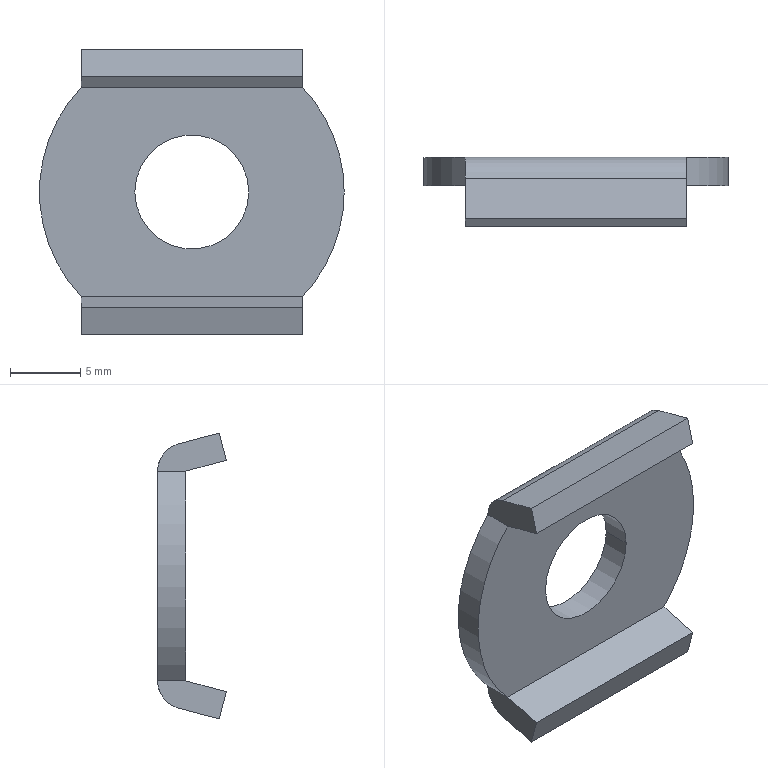Component | SolidWorks | CH-225-D-1_FW-516-1 | 1 solid | 19 faces | box 21.65 x 4.9 x 20.32 mm | volume 757 mm3 | plane 12 | cylinder 7 | commonest cylinder face diameters 21.645 x3 8.1 x2 4 x2
STEP:
#1=COLOUR_RGB('',0.7922,0.8196,0.9333);
#2=FILL_AREA_STYLE_COLOUR('',#1);
#3=FILL_AREA_STYLE('',(#2));
#4=SURFACE_STYLE_FILL_AREA(#3);
#5=SURFACE_SIDE_STYLE('',(#4));
#6=SURFACE_STYLE_USAGE(.BOTH.,#5);
#7=PRESENTATION_STYLE_ASSIGNMENT((#6));
#8=CARTESIAN_POINT('',(-1.339,3.61,4.64));
#9=VERTEX_POINT('',#8);
#10=CARTESIAN_POINT('',(-1.02,3.61,4.64));
#11=VERTEX_POINT('',#10);
#12=CARTESIAN_POINT('',(-1.179,3.61,4.64));
#13=DIRECTION('',(0.0001379,-1.,0.));
#14=DIRECTION('',(-1.,-0.0001379,0.));
#15=AXIS2_PLACEMENT_3D('',#12,#13,#14);
#16=CIRCLE('',#15,0.1594);
#17=EDGE_CURVE('',#9,#11,#16,.T.);
#18=ORIENTED_EDGE('',*,*,#17,.T.);
#19=CARTESIAN_POINT('',(-1.02,3.689,4.64));
#20=VERTEX_POINT('',#19);
#21=CARTESIAN_POINT('',(-1.02,3.61,4.64));
#22=DIRECTION('',(-0.0001379,1.,0.));
#23=VECTOR('',#22,39.37);
#24=LINE('',#21,#23);
#25=EDGE_CURVE('',#11,#20,#24,.T.);
#26=ORIENTED_EDGE('',*,*,#25,.T.);
#27=CARTESIAN_POINT('',(-1.339,3.689,4.64));
#28=VERTEX_POINT('',#27);
#29=CARTESIAN_POINT('',(-1.179,3.689,4.64));
#30=DIRECTION('',(-0.0001379,1.,0.));
#31=DIRECTION('',(-1.,-0.0001379,0.));
#32=AXIS2_PLACEMENT_3D('',#29,#30,#31);
#33=CIRCLE('',#32,0.1594);
#34=EDGE_CURVE('',#20,#28,#33,.T.);
#35=ORIENTED_EDGE('',*,*,#34,.T.);
#36=CARTESIAN_POINT('',(-1.339,3.61,4.64));
#37=DIRECTION('',(-0.0001379,1.,0.));
#38=VECTOR('',#37,39.37);
#39=LINE('',#36,#38);
#40=EDGE_CURVE('',#9,#28,#39,.T.);
#41=ORIENTED_EDGE('',*,*,#40,.F.);
#42=EDGE_LOOP('',(#18,#26,#35,#41));
#43=FACE_OUTER_BOUND('',#42,.T.);
#44=CARTESIAN_POINT('',(-1.179,3.61,4.64));
#45=DIRECTION('',(-0.0001379,1.,0.));
#46=DIRECTION('',(-1.,-0.0001379,0.));
#47=AXIS2_PLACEMENT_3D('',#44,#45,#46);
#48=CYLINDRICAL_SURFACE('',#47,0.1594);
#49=ADVANCED_FACE('',(#43),#48,.F.);
#50=CARTESIAN_POINT('',(-0.8702,3.689,4.346));
#51=VERTEX_POINT('',#50);
#52=CARTESIAN_POINT('',(-0.7532,3.689,4.64));
#53=VERTEX_POINT('',#52);
#54=CARTESIAN_POINT('',(-1.179,3.689,4.64));
#55=DIRECTION('',(0.0001379,-1.,0.));
#56=DIRECTION('',(1.,0.0001379,0.));
#57=AXIS2_PLACEMENT_3D('',#54,#55,#56);
#58=CIRCLE('',#57,0.4261);
#59=EDGE_CURVE('',#51,#53,#58,.T.);
#60=ORIENTED_EDGE('',*,*,#59,.T.);
#61=CARTESIAN_POINT('',(-0.7532,3.61,4.64));
#62=VERTEX_POINT('',#61);
#63=CARTESIAN_POINT('',(-0.7532,3.689,4.64));
#64=DIRECTION('',(0.0001379,-1.,0.));
#65=VECTOR('',#64,39.37);
#66=LINE('',#63,#65);
#67=EDGE_CURVE('',#53,#62,#66,.T.);
#68=ORIENTED_EDGE('',*,*,#67,.T.);
#69=CARTESIAN_POINT('',(-0.8702,3.61,4.346));
#70=VERTEX_POINT('',#69);
#71=CARTESIAN_POINT('',(-1.179,3.61,4.64));
#72=DIRECTION('',(-0.0001379,1.,-0.));
#73=DIRECTION('',(1.,0.0001379,0.));
#74=AXIS2_PLACEMENT_3D('',#71,#72,#73);
#75=CIRCLE('',#74,0.4261);
#76=EDGE_CURVE('',#62,#70,#75,.T.);
#77=ORIENTED_EDGE('',*,*,#76,.T.);
#78=CARTESIAN_POINT('',(-0.8702,3.649,4.346));
#79=DIRECTION('',(0.0001379,-1.,0.));
#80=VECTOR('',#79,39.37);
#81=LINE('',#78,#80);
#82=EDGE_CURVE('',#51,#70,#81,.T.);
#83=ORIENTED_EDGE('',*,*,#82,.F.);
#84=EDGE_LOOP('',(#60,#68,#77,#83));
#85=FACE_OUTER_BOUND('',#84,.T.);
#86=CARTESIAN_POINT('',(-1.179,3.689,4.64));
#87=DIRECTION('',(0.0001379,-1.,0.));
#88=DIRECTION('',(1.,0.0001379,0.));
#89=AXIS2_PLACEMENT_3D('',#86,#87,#88);
#90=CYLINDRICAL_SURFACE('',#89,0.4261);
#91=ADVANCED_FACE('',(#85),#90,.T.);
#92=ORIENTED_EDGE('',*,*,#25,.F.);
#93=CARTESIAN_POINT('',(-1.179,3.61,4.64));
#94=DIRECTION('',(0.0001379,-1.,0.));
#95=DIRECTION('',(-1.,-0.0001379,0.));
#96=AXIS2_PLACEMENT_3D('',#93,#94,#95);
#97=CIRCLE('',#96,0.1594);
#98=EDGE_CURVE('',#11,#9,#97,.T.);
#99=ORIENTED_EDGE('',*,*,#98,.T.);
#100=ORIENTED_EDGE('',*,*,#40,.T.);
#101=CARTESIAN_POINT('',(-1.179,3.689,4.64));
#102=DIRECTION('',(-0.0001379,1.,0.));
#103=DIRECTION('',(-1.,-0.0001379,0.));
#104=AXIS2_PLACEMENT_3D('',#101,#102,#103);
#105=CIRCLE('',#104,0.1594);
#106=EDGE_CURVE('',#28,#20,#105,.T.);
#107=ORIENTED_EDGE('',*,*,#106,.T.);
#108=EDGE_LOOP('',(#92,#99,#100,#107));
#109=FACE_OUTER_BOUND('',#108,.T.);
#110=CARTESIAN_POINT('',(-1.179,3.61,4.64));
#111=DIRECTION('',(-0.0001379,1.,0.));
#112=DIRECTION('',(-1.,-0.0001379,0.));
#113=AXIS2_PLACEMENT_3D('',#110,#111,#112);
#114=CYLINDRICAL_SURFACE('',#113,0.1594);
#115=ADVANCED_FACE('',(#109),#114,.F.);
#116=ORIENTED_EDGE('',*,*,#106,.F.);
#117=ORIENTED_EDGE('',*,*,#34,.F.);
#118=EDGE_LOOP('',(#116,#117));
#119=FACE_BOUND('',#118,.T.);
#120=ORIENTED_EDGE('',*,*,#59,.F.);
#121=CARTESIAN_POINT('',(-1.488,3.689,4.346));
#122=VERTEX_POINT('',#121);
#123=CARTESIAN_POINT('',(-1.179,3.689,4.346));
#124=DIRECTION('',(1.,0.0001379,0.));
#125=VECTOR('',#124,39.37);
#126=LINE('',#123,#125);
#127=EDGE_CURVE('',#122,#51,#126,.T.);
#128=ORIENTED_EDGE('',*,*,#127,.F.);
#129=CARTESIAN_POINT('',(-1.488,3.689,4.933));
#130=VERTEX_POINT('',#129);
#131=CARTESIAN_POINT('',(-1.179,3.689,4.64));
#132=DIRECTION('',(0.0001379,-1.,0.));
#133=DIRECTION('',(1.,0.0001379,0.));
#134=AXIS2_PLACEMENT_3D('',#131,#132,#133);
#135=CIRCLE('',#134,0.4261);
#136=EDGE_CURVE('',#130,#122,#135,.T.);
#137=ORIENTED_EDGE('',*,*,#136,.F.);
#138=CARTESIAN_POINT('',(-0.8702,3.689,4.933));
#139=VERTEX_POINT('',#138);
#140=CARTESIAN_POINT('',(-1.179,3.689,4.933));
#141=DIRECTION('',(-1.,-0.0001379,0.));
#142=VECTOR('',#141,39.37);
#143=LINE('',#140,#142);
#144=EDGE_CURVE('',#139,#130,#143,.T.);
#145=ORIENTED_EDGE('',*,*,#144,.F.);
#146=CARTESIAN_POINT('',(-1.179,3.689,4.64));
#147=DIRECTION('',(0.0001379,-1.,0.));
#148=DIRECTION('',(1.,0.0001379,0.));
#149=AXIS2_PLACEMENT_3D('',#146,#147,#148);
#150=CIRCLE('',#149,0.4261);
#151=EDGE_CURVE('',#53,#139,#150,.T.);
#152=ORIENTED_EDGE('',*,*,#151,.F.);
#153=EDGE_LOOP('',(#120,#128,#137,#145,#152));
#154=FACE_OUTER_BOUND('',#153,.T.);
#155=CARTESIAN_POINT('',(-1.61,3.689,4.346));
#156=DIRECTION('',(0.0001379,-1.,0.));
#157=DIRECTION('',(1.,0.0001379,0.));
#158=AXIS2_PLACEMENT_3D('',#155,#156,#157);
#159=PLANE('',#158);
#160=ADVANCED_FACE('',(#119,#154),#159,.F.);
#161=ORIENTED_EDGE('',*,*,#17,.F.);
#162=ORIENTED_EDGE('',*,*,#98,.F.);
#163=EDGE_LOOP('',(#161,#162));
#164=FACE_BOUND('',#163,.T.);
#165=CARTESIAN_POINT('',(-0.8702,3.61,4.933));
#166=VERTEX_POINT('',#165);
#167=CARTESIAN_POINT('',(-1.179,3.61,4.64));
#168=DIRECTION('',(-0.0001379,1.,-0.));
#169=DIRECTION('',(1.,0.0001379,0.));
#170=AXIS2_PLACEMENT_3D('',#167,#168,#169);
#171=CIRCLE('',#170,0.4261);
#172=EDGE_CURVE('',#166,#62,#171,.T.);
#173=ORIENTED_EDGE('',*,*,#172,.F.);
#174=CARTESIAN_POINT('',(-1.488,3.61,4.933));
#175=VERTEX_POINT('',#174);
#176=CARTESIAN_POINT('',(-1.179,3.61,4.933));
#177=DIRECTION('',(1.,0.0001379,0.));
#178=VECTOR('',#177,39.37);
#179=LINE('',#176,#178);
#180=EDGE_CURVE('',#175,#166,#179,.T.);
#181=ORIENTED_EDGE('',*,*,#180,.F.);
#182=CARTESIAN_POINT('',(-1.488,3.61,4.346));
#183=VERTEX_POINT('',#182);
#184=CARTESIAN_POINT('',(-1.179,3.61,4.64));
#185=DIRECTION('',(-0.0001379,1.,-0.));
#186=DIRECTION('',(1.,0.0001379,-0.));
#187=AXIS2_PLACEMENT_3D('',#184,#185,#186);
#188=CIRCLE('',#187,0.4261);
#189=EDGE_CURVE('',#183,#175,#188,.T.);
#190=ORIENTED_EDGE('',*,*,#189,.F.);
#191=CARTESIAN_POINT('',(-1.179,3.61,4.346));
#192=DIRECTION('',(-1.,-0.0001379,0.));
#193=VECTOR('',#192,39.37);
#194=LINE('',#191,#193);
#195=EDGE_CURVE('',#70,#183,#194,.T.);
#196=ORIENTED_EDGE('',*,*,#195,.F.);
#197=ORIENTED_EDGE('',*,*,#76,.F.);
#198=EDGE_LOOP('',(#173,#181,#190,#196,#197));
#199=FACE_OUTER_BOUND('',#198,.T.);
#200=CARTESIAN_POINT('',(-0.7481,3.61,4.933));
#201=DIRECTION('',(-0.0001379,1.,0.));
#202=DIRECTION('',(0.,0.,-1.));
#203=AXIS2_PLACEMENT_3D('',#200,#201,#202);
#204=PLANE('',#203);
#205=ADVANCED_FACE('',(#164,#199),#204,.F.);
#206=ORIENTED_EDGE('',*,*,#144,.T.);
#207=CARTESIAN_POINT('',(-1.488,3.63,5.009));
#208=VERTEX_POINT('',#207);
#209=CARTESIAN_POINT('',(-1.488,3.61,4.933));
#210=DIRECTION('',(-1.,-0.0001379,0.));
#211=DIRECTION('',(-0.0001379,1.,-0.));
#212=AXIS2_PLACEMENT_3D('',#209,#210,#211);
#213=CIRCLE('',#212,0.07874);
#214=EDGE_CURVE('',#208,#130,#213,.T.);
#215=ORIENTED_EDGE('',*,*,#214,.F.);
#216=CARTESIAN_POINT('',(-0.8702,3.63,5.009));
#217=VERTEX_POINT('',#216);
#218=CARTESIAN_POINT('',(-1.179,3.63,5.009));
#219=DIRECTION('',(-1.,-0.0001379,0.));
#220=VECTOR('',#219,39.37);
#221=LINE('',#218,#220);
#222=EDGE_CURVE('',#217,#208,#221,.T.);
#223=ORIENTED_EDGE('',*,*,#222,.F.);
#224=CARTESIAN_POINT('',(-0.8702,3.61,4.933));
#225=DIRECTION('',(1.,0.0001379,-0.));
#226=DIRECTION('',(-0.0001379,1.,0.));
#227=AXIS2_PLACEMENT_3D('',#224,#225,#226);
#228=CIRCLE('',#227,0.07874);
#229=EDGE_CURVE('',#139,#217,#228,.T.);
#230=ORIENTED_EDGE('',*,*,#229,.F.);
#231=EDGE_LOOP('',(#206,#215,#223,#230));
#232=FACE_OUTER_BOUND('',#231,.T.);
#233=CARTESIAN_POINT('',(-1.488,3.61,4.933));
#234=DIRECTION('',(1.,0.0001379,-0.));
#235=DIRECTION('',(-0.0001379,1.,0.));
#236=AXIS2_PLACEMENT_3D('',#233,#234,#235);
#237=CYLINDRICAL_SURFACE('',#236,0.07874);
#238=ADVANCED_FACE('',(#232),#237,.T.);
#239=ORIENTED_EDGE('',*,*,#67,.F.);
#240=ORIENTED_EDGE('',*,*,#151,.T.);
#241=CARTESIAN_POINT('',(-0.8702,3.649,4.933));
#242=DIRECTION('',(-0.0001379,1.,0.));
#243=VECTOR('',#242,39.37);
#244=LINE('',#241,#243);
#245=EDGE_CURVE('',#166,#139,#244,.T.);
#246=ORIENTED_EDGE('',*,*,#245,.F.);
#247=ORIENTED_EDGE('',*,*,#172,.T.);
#248=EDGE_LOOP('',(#239,#240,#246,#247));
#249=FACE_OUTER_BOUND('',#248,.T.);
#250=CARTESIAN_POINT('',(-1.179,3.689,4.64));
#251=DIRECTION('',(0.0001379,-1.,0.));
#252=DIRECTION('',(1.,0.0001379,0.));
#253=AXIS2_PLACEMENT_3D('',#250,#251,#252);
#254=CYLINDRICAL_SURFACE('',#253,0.4261);
#255=ADVANCED_FACE('',(#249),#254,.T.);
#256=CARTESIAN_POINT('',(-0.8702,3.63,4.27));
#257=VERTEX_POINT('',#256);
#258=CARTESIAN_POINT('',(-0.8702,3.61,4.346));
#259=DIRECTION('',(1.,0.0001379,0.));
#260=DIRECTION('',(-0.0001379,1.,0.));
#261=AXIS2_PLACEMENT_3D('',#258,#259,#260);
#262=CIRCLE('',#261,0.07874);
#263=EDGE_CURVE('',#257,#51,#262,.T.);
#264=ORIENTED_EDGE('',*,*,#263,.F.);
#265=CARTESIAN_POINT('',(-1.488,3.63,4.27));
#266=VERTEX_POINT('',#265);
#267=CARTESIAN_POINT('',(-1.179,3.63,4.27));
#268=DIRECTION('',(1.,0.0001379,0.));
#269=VECTOR('',#268,39.37);
#270=LINE('',#267,#269);
#271=EDGE_CURVE('',#266,#257,#270,.T.);
#272=ORIENTED_EDGE('',*,*,#271,.F.);
#273=CARTESIAN_POINT('',(-1.488,3.61,4.346));
#274=DIRECTION('',(-1.,-0.0001379,0.));
#275=DIRECTION('',(-0.0001379,1.,-0.));
#276=AXIS2_PLACEMENT_3D('',#273,#274,#275);
#277=CIRCLE('',#276,0.07874);
#278=EDGE_CURVE('',#122,#266,#277,.T.);
#279=ORIENTED_EDGE('',*,*,#278,.F.);
#280=ORIENTED_EDGE('',*,*,#127,.T.);
#281=EDGE_LOOP('',(#264,#272,#279,#280));
#282=FACE_OUTER_BOUND('',#281,.T.);
#283=CARTESIAN_POINT('',(-1.488,3.61,4.346));
#284=DIRECTION('',(1.,0.0001379,0.));
#285=DIRECTION('',(-0.0001379,1.,0.));
#286=AXIS2_PLACEMENT_3D('',#283,#284,#285);
#287=CYLINDRICAL_SURFACE('',#286,0.07874);
#288=ADVANCED_FACE('',(#282),#287,.T.);
#289=ORIENTED_EDGE('',*,*,#189,.T.);
#290=CARTESIAN_POINT('',(-1.488,3.649,4.933));
#291=DIRECTION('',(0.0001379,-1.,0.));
#292=VECTOR('',#291,39.37);
#293=LINE('',#290,#292);
#294=EDGE_CURVE('',#130,#175,#293,.T.);
#295=ORIENTED_EDGE('',*,*,#294,.F.);
#296=ORIENTED_EDGE('',*,*,#136,.T.);
#297=CARTESIAN_POINT('',(-1.488,3.649,4.346));
#298=DIRECTION('',(-0.0001379,1.,0.));
#299=VECTOR('',#298,39.37);
#300=LINE('',#297,#299);
#301=EDGE_CURVE('',#183,#122,#300,.T.);
#302=ORIENTED_EDGE('',*,*,#301,.F.);
#303=EDGE_LOOP('',(#289,#295,#296,#302));
#304=FACE_OUTER_BOUND('',#303,.T.);
#305=CARTESIAN_POINT('',(-1.179,3.689,4.64));
#306=DIRECTION('',(0.0001379,-1.,0.));
#307=DIRECTION('',(1.,0.0001379,0.));
#308=AXIS2_PLACEMENT_3D('',#305,#306,#307);
#309=CYLINDRICAL_SURFACE('',#308,0.4261);
#310=ADVANCED_FACE('',(#304),#309,.T.);
#311=ORIENTED_EDGE('',*,*,#195,.T.);
#312=CARTESIAN_POINT('',(-1.488,3.496,4.316));
#313=VERTEX_POINT('',#312);
#314=CARTESIAN_POINT('',(-1.488,3.553,4.331));
#315=DIRECTION('',(-0.0001332,0.9659,0.2588));
#316=VECTOR('',#315,39.37);
#317=LINE('',#314,#316);
#318=EDGE_CURVE('',#313,#183,#317,.T.);
#319=ORIENTED_EDGE('',*,*,#318,.F.);
#320=CARTESIAN_POINT('',(-0.8702,3.496,4.316));
#321=VERTEX_POINT('',#320);
#322=CARTESIAN_POINT('',(-1.179,3.496,4.316));
#323=DIRECTION('',(-1.,-0.0001379,0.));
#324=VECTOR('',#323,39.37);
#325=LINE('',#322,#324);
#326=EDGE_CURVE('',#321,#313,#325,.T.);
#327=ORIENTED_EDGE('',*,*,#326,.F.);
#328=CARTESIAN_POINT('',(-0.8702,3.553,4.331));
#329=DIRECTION('',(0.0001332,-0.9659,-0.2588));
#330=VECTOR('',#329,39.37);
#331=LINE('',#328,#330);
#332=EDGE_CURVE('',#70,#321,#331,.T.);
#333=ORIENTED_EDGE('',*,*,#332,.F.);
#334=EDGE_LOOP('',(#311,#319,#327,#333));
#335=FACE_OUTER_BOUND('',#334,.T.);
#336=CARTESIAN_POINT('',(-0.8702,3.61,4.346));
#337=DIRECTION('',(-0.00003569,0.2588,-0.9659));
#338=DIRECTION('',(0.0001332,-0.9659,-0.2588));
#339=AXIS2_PLACEMENT_3D('',#336,#337,#338);
#340=PLANE('',#339);
#341=ADVANCED_FACE('',(#335),#340,.F.);
#342=CARTESIAN_POINT('',(-0.8702,3.496,4.963));
#343=VERTEX_POINT('',#342);
#344=CARTESIAN_POINT('',(-0.8702,3.553,4.948));
#345=DIRECTION('',(-0.0001332,0.9659,-0.2588));
#346=VECTOR('',#345,39.37);
#347=LINE('',#344,#346);
#348=EDGE_CURVE('',#343,#166,#347,.T.);
#349=ORIENTED_EDGE('',*,*,#348,.F.);
#350=CARTESIAN_POINT('',(-1.488,3.496,4.963));
#351=VERTEX_POINT('',#350);
#352=CARTESIAN_POINT('',(-1.179,3.496,4.963));
#353=DIRECTION('',(1.,0.0001379,0.));
#354=VECTOR('',#353,39.37);
#355=LINE('',#352,#354);
#356=EDGE_CURVE('',#351,#343,#355,.T.);
#357=ORIENTED_EDGE('',*,*,#356,.F.);
#358=CARTESIAN_POINT('',(-1.488,3.553,4.948));
#359=DIRECTION('',(0.0001332,-0.9659,0.2588));
#360=VECTOR('',#359,39.37);
#361=LINE('',#358,#360);
#362=EDGE_CURVE('',#175,#351,#361,.T.);
#363=ORIENTED_EDGE('',*,*,#362,.F.);
#364=ORIENTED_EDGE('',*,*,#180,.T.);
#365=EDGE_LOOP('',(#349,#357,#363,#364));
#366=FACE_OUTER_BOUND('',#365,.T.);
#367=CARTESIAN_POINT('',(-0.8702,3.496,4.963));
#368=DIRECTION('',(-0.00003569,0.2588,0.9659));
#369=DIRECTION('',(-0.0001332,0.9659,-0.2588));
#370=AXIS2_PLACEMENT_3D('',#367,#368,#369);
#371=PLANE('',#370);
#372=ADVANCED_FACE('',(#366),#371,.F.);
#373=ORIENTED_EDGE('',*,*,#245,.T.);
#374=ORIENTED_EDGE('',*,*,#229,.T.);
#375=CARTESIAN_POINT('',(-0.8702,3.516,5.039));
#376=VERTEX_POINT('',#375);
#377=CARTESIAN_POINT('',(-0.8702,3.63,5.009));
#378=DIRECTION('',(-0.0001332,0.9659,-0.2588));
#379=VECTOR('',#378,39.37);
#380=LINE('',#377,#379);
#381=EDGE_CURVE('',#376,#217,#380,.T.);
#382=ORIENTED_EDGE('',*,*,#381,.F.);
#383=CARTESIAN_POINT('',(-0.8702,3.516,5.039));
#384=DIRECTION('',(-0.00003569,0.2588,0.9659));
#385=VECTOR('',#384,39.37);
#386=LINE('',#383,#385);
#387=EDGE_CURVE('',#343,#376,#386,.T.);
#388=ORIENTED_EDGE('',*,*,#387,.F.);
#389=ORIENTED_EDGE('',*,*,#348,.T.);
#390=EDGE_LOOP('',(#373,#374,#382,#388,#389));
#391=FACE_OUTER_BOUND('',#390,.T.);
#392=CARTESIAN_POINT('',(-0.8702,3.495,4.933));
#393=DIRECTION('',(-1.,-0.0001379,0.));
#394=DIRECTION('',(0.,0.,1.));
#395=AXIS2_PLACEMENT_3D('',#392,#393,#394);
#396=PLANE('',#395);
#397=ADVANCED_FACE('',(#391),#396,.F.);
#398=CARTESIAN_POINT('',(-1.488,3.516,5.039));
#399=VERTEX_POINT('',#398);
#400=CARTESIAN_POINT('',(-1.488,3.63,5.009));
#401=DIRECTION('',(0.0001332,-0.9659,0.2588));
#402=VECTOR('',#401,39.37);
#403=LINE('',#400,#402);
#404=EDGE_CURVE('',#208,#399,#403,.T.);
#405=ORIENTED_EDGE('',*,*,#404,.F.);
#406=ORIENTED_EDGE('',*,*,#214,.T.);
#407=ORIENTED_EDGE('',*,*,#294,.T.);
#408=ORIENTED_EDGE('',*,*,#362,.T.);
#409=CARTESIAN_POINT('',(-1.488,3.516,5.039));
#410=DIRECTION('',(0.00003569,-0.2588,-0.9659));
#411=VECTOR('',#410,39.37);
#412=LINE('',#409,#411);
#413=EDGE_CURVE('',#399,#351,#412,.T.);
#414=ORIENTED_EDGE('',*,*,#413,.F.);
#415=EDGE_LOOP('',(#405,#406,#407,#408,#414));
#416=FACE_OUTER_BOUND('',#415,.T.);
#417=CARTESIAN_POINT('',(-1.488,3.495,5.04));
#418=DIRECTION('',(1.,0.0001379,0.));
#419=DIRECTION('',(0.,0.,-1.));
#420=AXIS2_PLACEMENT_3D('',#417,#418,#419);
#421=PLANE('',#420);
#422=ADVANCED_FACE('',(#416),#421,.F.);
#423=ORIENTED_EDGE('',*,*,#404,.T.);
#424=CARTESIAN_POINT('',(-1.179,3.516,5.039));
#425=DIRECTION('',(-1.,-0.0001379,0.));
#426=VECTOR('',#425,39.37);
#427=LINE('',#424,#426);
#428=EDGE_CURVE('',#376,#399,#427,.T.);
#429=ORIENTED_EDGE('',*,*,#428,.F.);
#430=ORIENTED_EDGE('',*,*,#381,.T.);
#431=ORIENTED_EDGE('',*,*,#222,.T.);
#432=EDGE_LOOP('',(#423,#429,#430,#431));
#433=FACE_OUTER_BOUND('',#432,.T.);
#434=CARTESIAN_POINT('',(-0.8702,3.63,5.009));
#435=DIRECTION('',(0.00003569,-0.2588,-0.9659));
#436=DIRECTION('',(0.0001332,-0.9659,0.2588));
#437=AXIS2_PLACEMENT_3D('',#434,#435,#436);
#438=PLANE('',#437);
#439=ADVANCED_FACE('',(#433),#438,.F.);
#440=ORIENTED_EDGE('',*,*,#82,.T.);
#441=ORIENTED_EDGE('',*,*,#332,.T.);
#442=CARTESIAN_POINT('',(-0.8702,3.516,4.24));
#443=VERTEX_POINT('',#442);
#444=CARTESIAN_POINT('',(-0.8702,3.496,4.316));
#445=DIRECTION('',(0.00003569,-0.2588,0.9659));
#446=VECTOR('',#445,39.37);
#447=LINE('',#444,#446);
#448=EDGE_CURVE('',#443,#321,#447,.T.);
#449=ORIENTED_EDGE('',*,*,#448,.F.);
#450=CARTESIAN_POINT('',(-0.8702,3.516,4.24));
#451=DIRECTION('',(0.0001332,-0.9659,-0.2588));
#452=VECTOR('',#451,39.37);
#453=LINE('',#450,#452);
#454=EDGE_CURVE('',#257,#443,#453,.T.);
#455=ORIENTED_EDGE('',*,*,#454,.F.);
#456=ORIENTED_EDGE('',*,*,#263,.T.);
#457=EDGE_LOOP('',(#440,#441,#449,#455,#456));
#458=FACE_OUTER_BOUND('',#457,.T.);
#459=CARTESIAN_POINT('',(-0.8702,3.495,4.239));
#460=DIRECTION('',(-1.,-0.0001379,0.));
#461=DIRECTION('',(0.,0.,1.));
#462=AXIS2_PLACEMENT_3D('',#459,#460,#461);
#463=PLANE('',#462);
#464=ADVANCED_FACE('',(#458),#463,.F.);
#465=CARTESIAN_POINT('',(-1.488,3.516,4.24));
#466=VERTEX_POINT('',#465);
#467=CARTESIAN_POINT('',(-1.488,3.573,4.255));
#468=DIRECTION('',(0.0001332,-0.9659,-0.2588));
#469=VECTOR('',#468,39.37);
#470=LINE('',#467,#469);
#471=EDGE_CURVE('',#266,#466,#470,.T.);
#472=ORIENTED_EDGE('',*,*,#471,.F.);
#473=ORIENTED_EDGE('',*,*,#271,.T.);
#474=ORIENTED_EDGE('',*,*,#454,.T.);
#475=CARTESIAN_POINT('',(-1.179,3.516,4.24));
#476=DIRECTION('',(1.,0.0001379,0.));
#477=VECTOR('',#476,39.37);
#478=LINE('',#475,#477);
#479=EDGE_CURVE('',#466,#443,#478,.T.);
#480=ORIENTED_EDGE('',*,*,#479,.F.);
#481=EDGE_LOOP('',(#472,#473,#474,#480));
#482=FACE_OUTER_BOUND('',#481,.T.);
#483=CARTESIAN_POINT('',(-0.8702,3.516,4.24));
#484=DIRECTION('',(0.00003569,-0.2588,0.9659));
#485=DIRECTION('',(-0.0001332,0.9659,0.2588));
#486=AXIS2_PLACEMENT_3D('',#483,#484,#485);
#487=PLANE('',#486);
#488=ADVANCED_FACE('',(#482),#487,.F.);
#489=ORIENTED_EDGE('',*,*,#278,.T.);
#490=ORIENTED_EDGE('',*,*,#471,.T.);
#491=CARTESIAN_POINT('',(-1.488,3.496,4.316));
#492=DIRECTION('',(-0.00003569,0.2588,-0.9659));
#493=VECTOR('',#492,39.37);
#494=LINE('',#491,#493);
#495=EDGE_CURVE('',#313,#466,#494,.T.);
#496=ORIENTED_EDGE('',*,*,#495,.F.);
#497=ORIENTED_EDGE('',*,*,#318,.T.);
#498=ORIENTED_EDGE('',*,*,#301,.T.);
#499=EDGE_LOOP('',(#489,#490,#496,#497,#498));
#500=FACE_OUTER_BOUND('',#499,.T.);
#501=CARTESIAN_POINT('',(-1.488,3.495,4.346));
#502=DIRECTION('',(1.,0.0001379,0.));
#503=DIRECTION('',(0.,0.,-1.));
#504=AXIS2_PLACEMENT_3D('',#501,#502,#503);
#505=PLANE('',#504);
#506=ADVANCED_FACE('',(#500),#505,.F.);
#507=ORIENTED_EDGE('',*,*,#495,.T.);
#508=ORIENTED_EDGE('',*,*,#479,.T.);
#509=ORIENTED_EDGE('',*,*,#448,.T.);
#510=ORIENTED_EDGE('',*,*,#326,.T.);
#511=EDGE_LOOP('',(#507,#508,#509,#510));
#512=FACE_OUTER_BOUND('',#511,.T.);
#513=CARTESIAN_POINT('',(-0.8702,3.496,4.316));
#514=DIRECTION('',(-0.0001332,0.9659,0.2588));
#515=DIRECTION('',(-0.00003569,0.2588,-0.9659));
#516=AXIS2_PLACEMENT_3D('',#513,#514,#515);
#517=PLANE('',#516);
#518=ADVANCED_FACE('',(#512),#517,.F.);
#519=ORIENTED_EDGE('',*,*,#413,.T.);
#520=ORIENTED_EDGE('',*,*,#356,.T.);
#521=ORIENTED_EDGE('',*,*,#387,.T.);
#522=ORIENTED_EDGE('',*,*,#428,.T.);
#523=EDGE_LOOP('',(#519,#520,#521,#522));
#524=FACE_OUTER_BOUND('',#523,.T.);
#525=CARTESIAN_POINT('',(-0.8702,3.516,5.039));
#526=DIRECTION('',(-0.0001332,0.9659,-0.2588));
#527=DIRECTION('',(0.00003569,-0.2588,-0.9659));
#528=AXIS2_PLACEMENT_3D('',#525,#526,#527);
#529=PLANE('',#528);
#530=ADVANCED_FACE('',(#524),#529,.F.);
#531=CLOSED_SHELL('',(#49,#91,#115,#160,#205,#238,#255,#288,#310,#341,#372,#397,#422,#439,#464,#488,#506,#518,#530));
#532=MANIFOLD_SOLID_BREP('',#531);
#533=STYLED_ITEM('',(#7),#532);
#534=(LENGTH_UNIT()NAMED_UNIT(*)SI_UNIT($,.METRE.));
#535=LENGTH_MEASURE_WITH_UNIT(LENGTH_MEASURE(0.0254),#534);
#536=DIMENSIONAL_EXPONENTS(1.,0.,0.,0.,0.,0.,0.);
#537=(CONVERSION_BASED_UNIT('',#535)LENGTH_UNIT()NAMED_UNIT(#536));
#538=UNCERTAINTY_MEASURE_WITH_UNIT(LENGTH_MEASURE(0.00001),#537,'','');
#539=(NAMED_UNIT(*)PLANE_ANGLE_UNIT()SI_UNIT($,.RADIAN.));
#540=(NAMED_UNIT(*)SI_UNIT($,.STERADIAN.)SOLID_ANGLE_UNIT());
#541=(GEOMETRIC_REPRESENTATION_CONTEXT(3)GLOBAL_UNCERTAINTY_ASSIGNED_CONTEXT((#538))GLOBAL_UNIT_ASSIGNED_CONTEXT((#537,#539,#540))REPRESENTATION_CONTEXT('',''));
#542=MECHANICAL_DESIGN_GEOMETRIC_PRESENTATION_REPRESENTATION('',(#533),#541);
#543=PRESENTATION_LAYER_ASSIGNMENT('','',(#533));
#544=CARTESIAN_POINT('',(0.,0.,0.));
#545=DIRECTION('',(0.,0.,1.));
#546=DIRECTION('',(1.,0.,0.));
#547=AXIS2_PLACEMENT_3D('',#544,#545,#546);
#548=(LENGTH_UNIT()NAMED_UNIT(*)SI_UNIT($,.METRE.));
#549=LENGTH_MEASURE_WITH_UNIT(LENGTH_MEASURE(0.0254),#548);
#550=DIMENSIONAL_EXPONENTS(1.,0.,0.,0.,0.,0.,0.);
#551=(CONVERSION_BASED_UNIT('',#549)LENGTH_UNIT()NAMED_UNIT(#550));
#552=UNCERTAINTY_MEASURE_WITH_UNIT(LENGTH_MEASURE(0.00001),#551,'','');
#553=(NAMED_UNIT(*)PLANE_ANGLE_UNIT()SI_UNIT($,.RADIAN.));
#554=(NAMED_UNIT(*)SI_UNIT($,.STERADIAN.)SOLID_ANGLE_UNIT());
#555=(GEOMETRIC_REPRESENTATION_CONTEXT(3)GLOBAL_UNCERTAINTY_ASSIGNED_CONTEXT((#552))GLOBAL_UNIT_ASSIGNED_CONTEXT((#551,#553,#554))REPRESENTATION_CONTEXT('',''));
#556=ADVANCED_BREP_SHAPE_REPRESENTATION('',(#532,#547),#555);